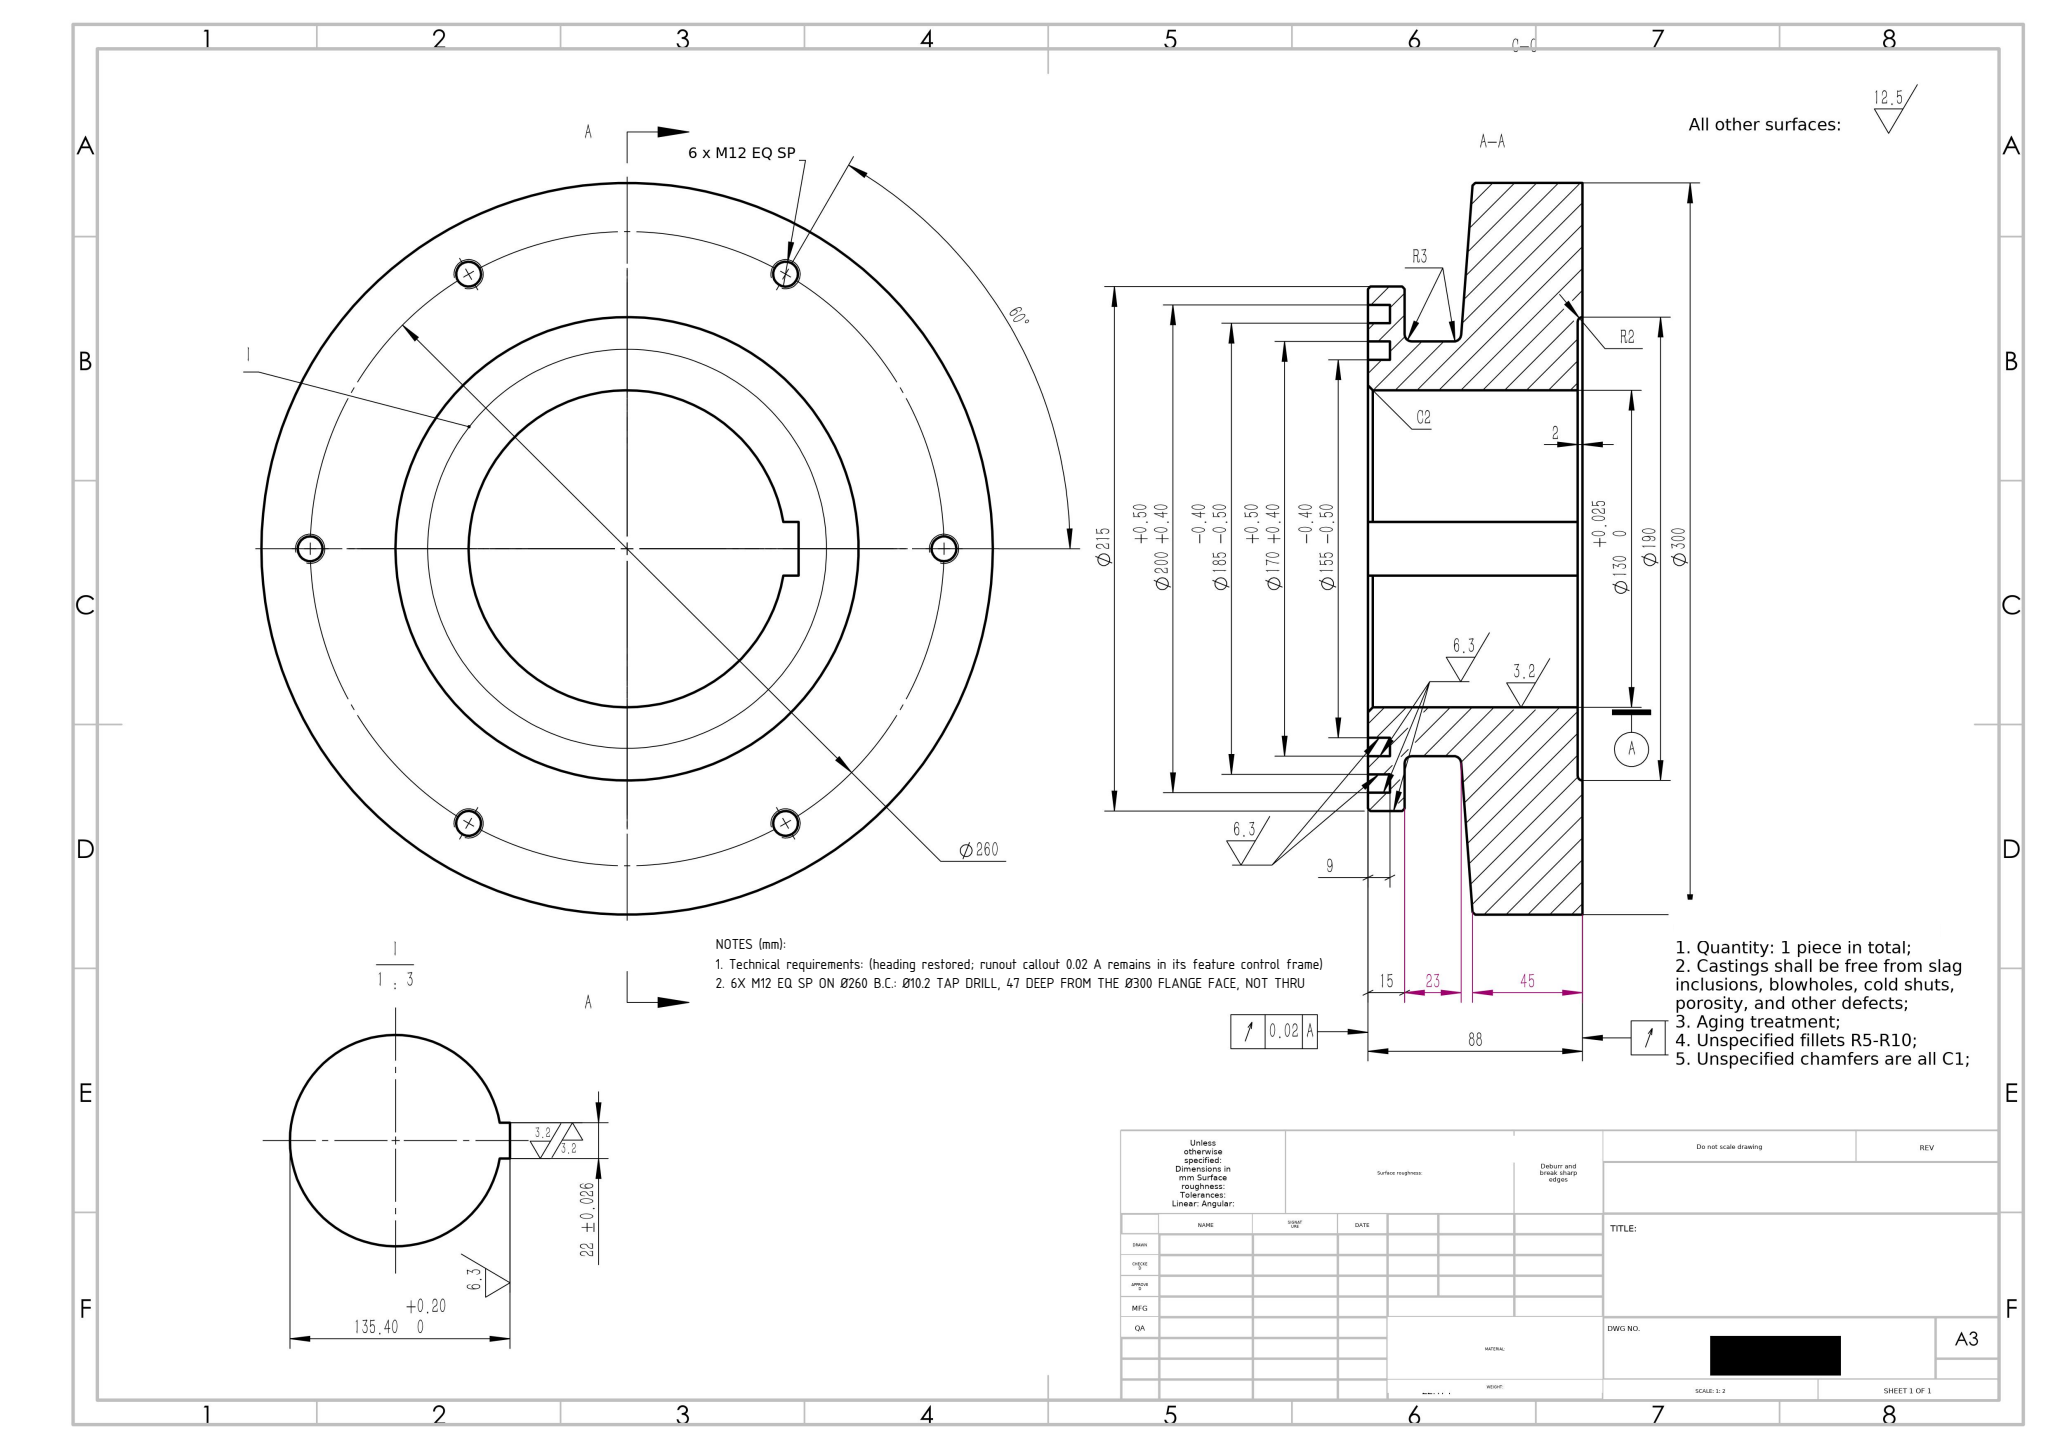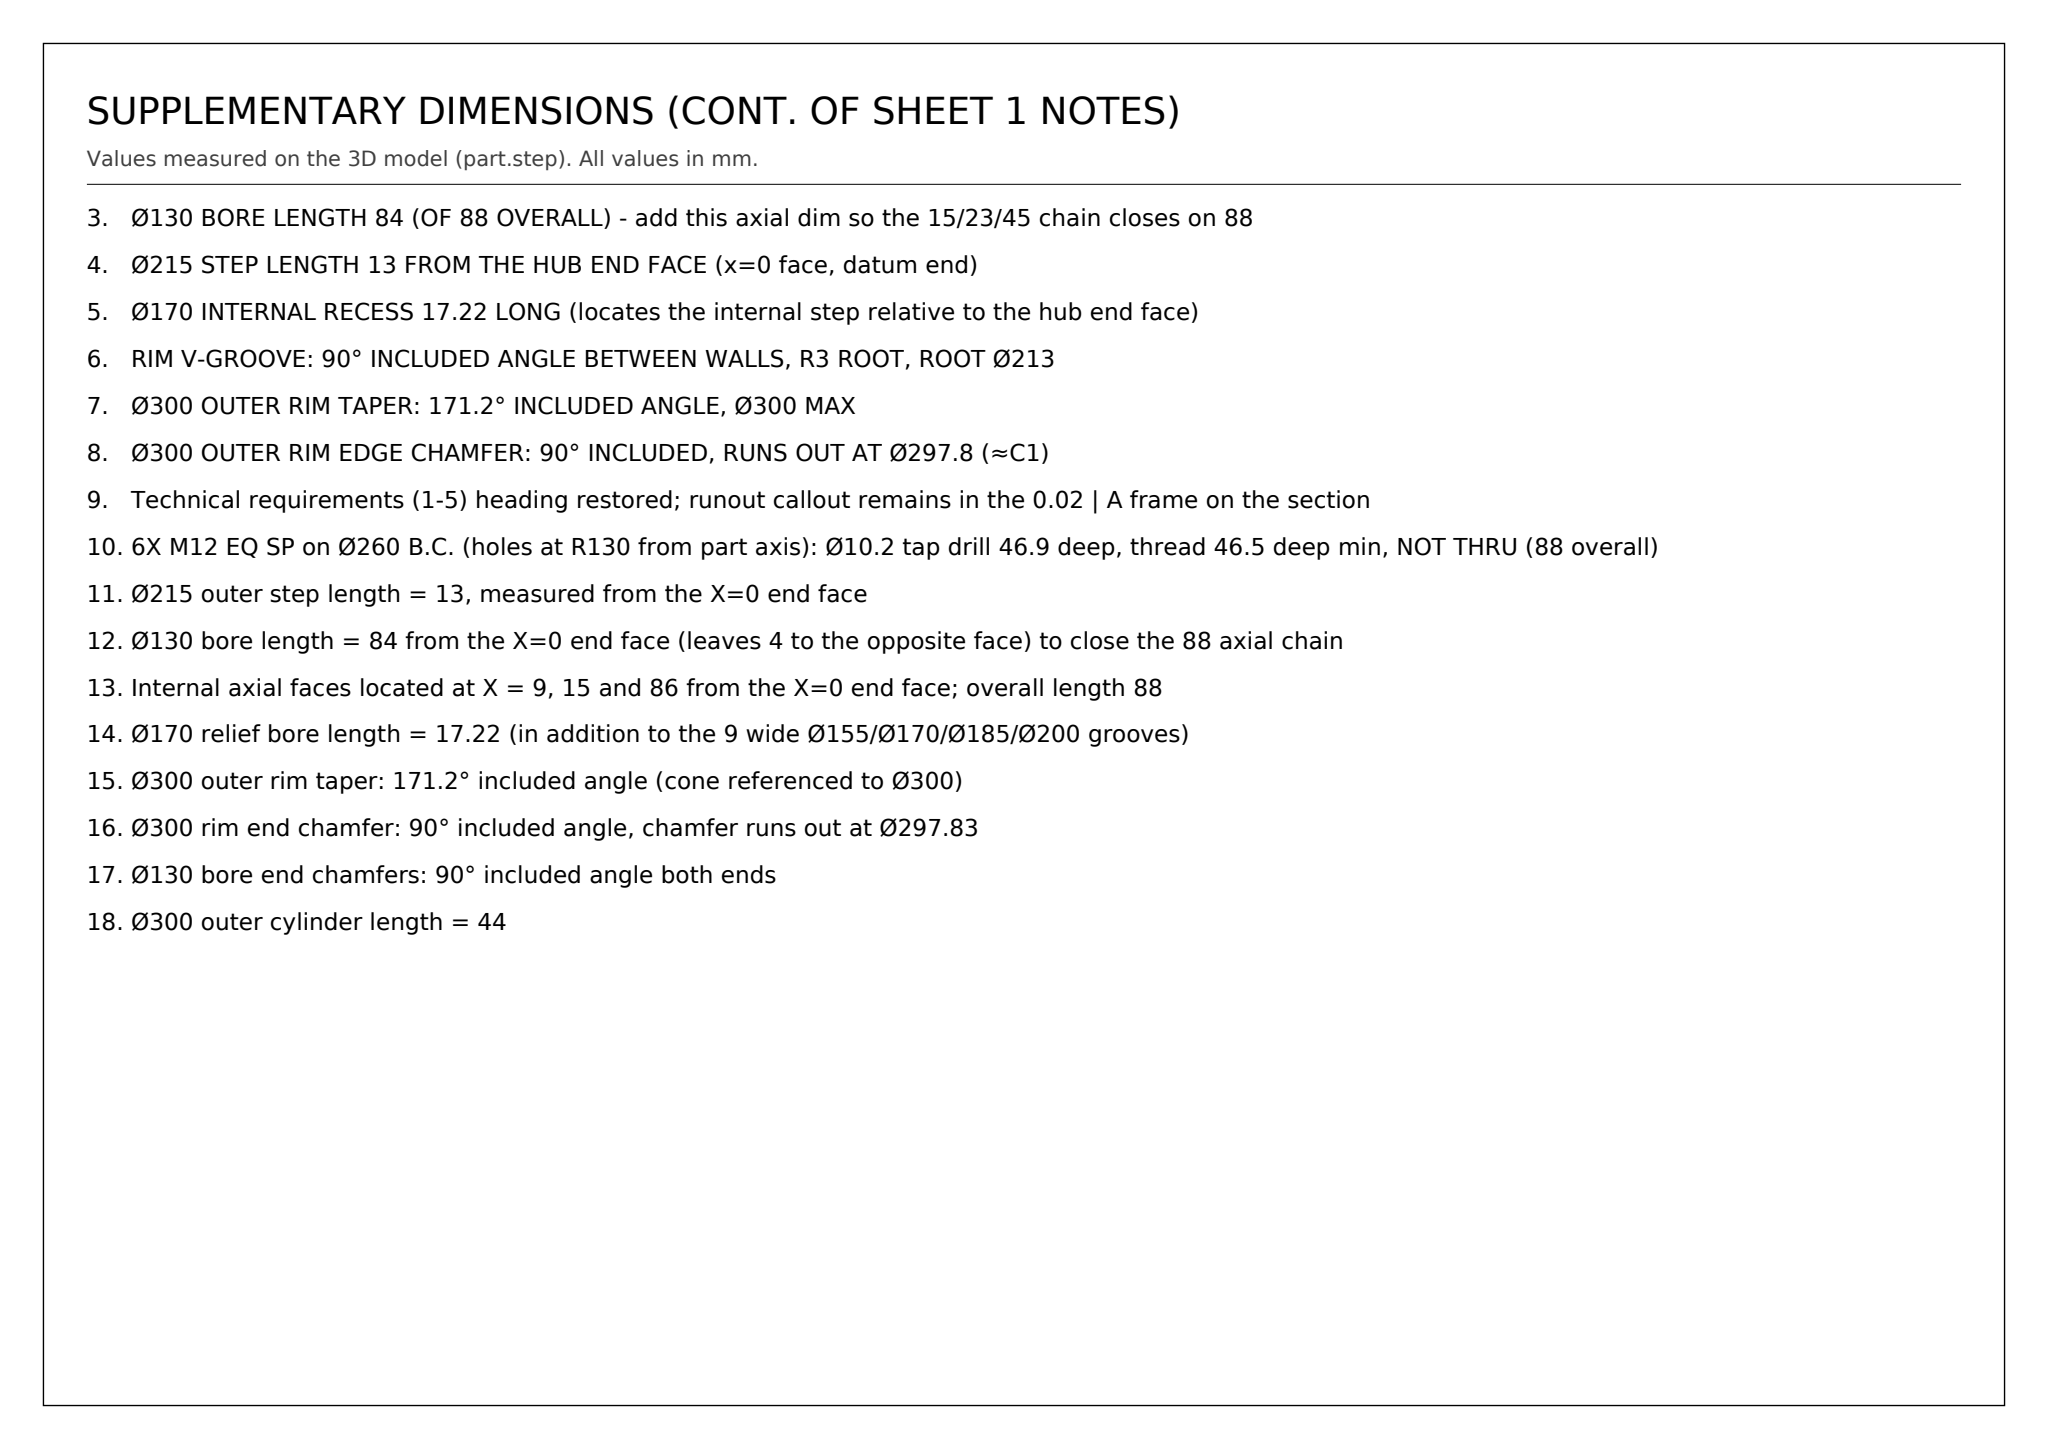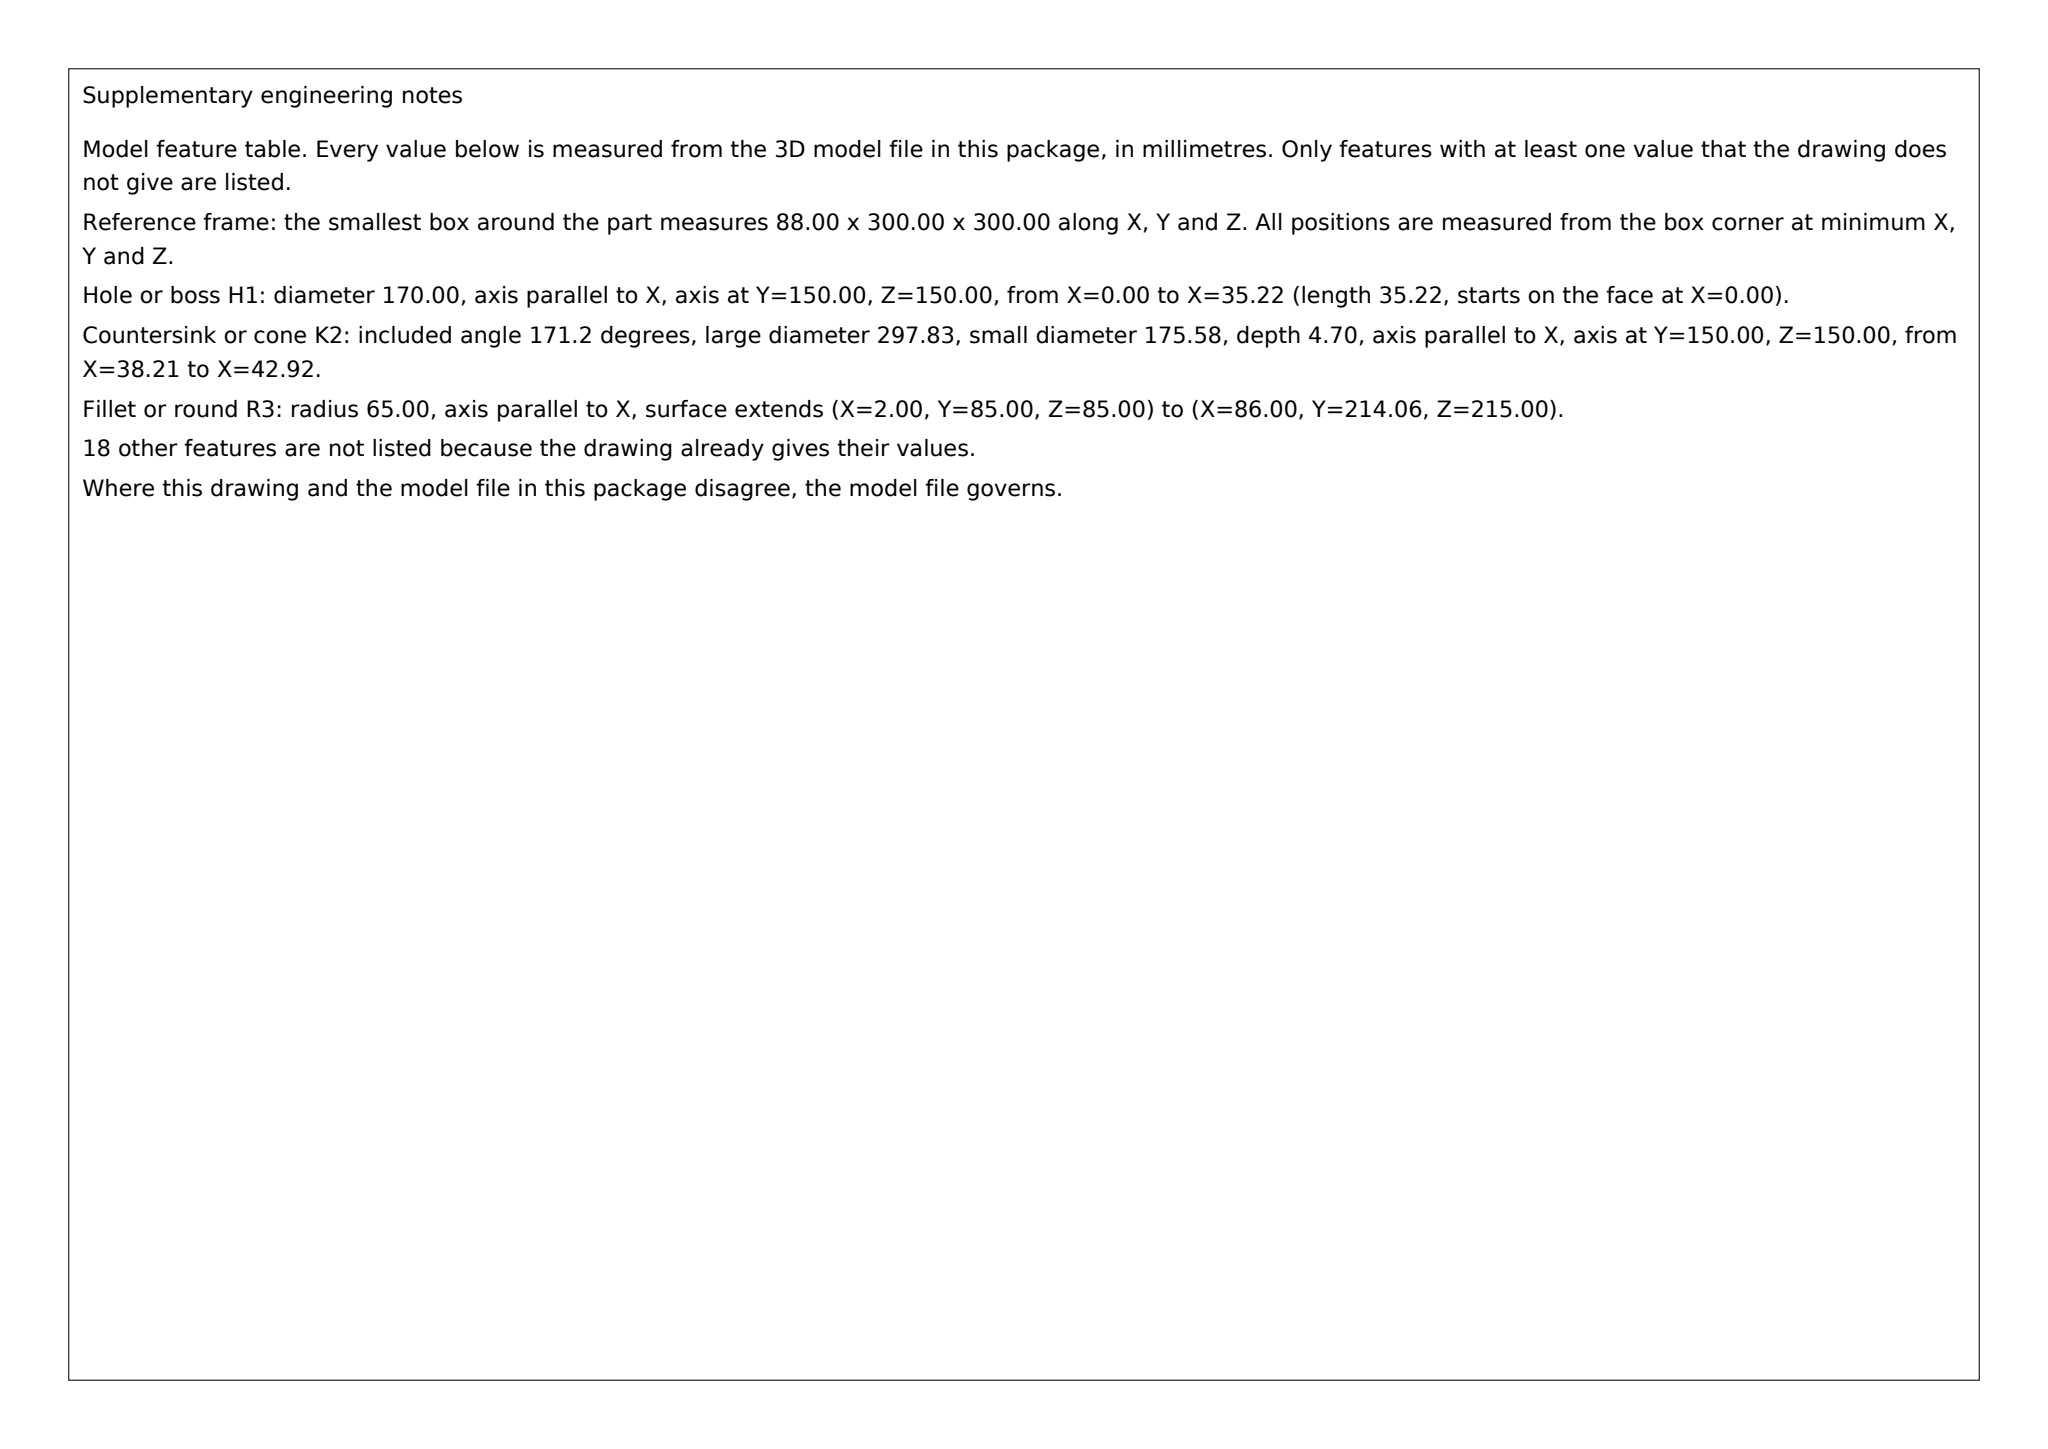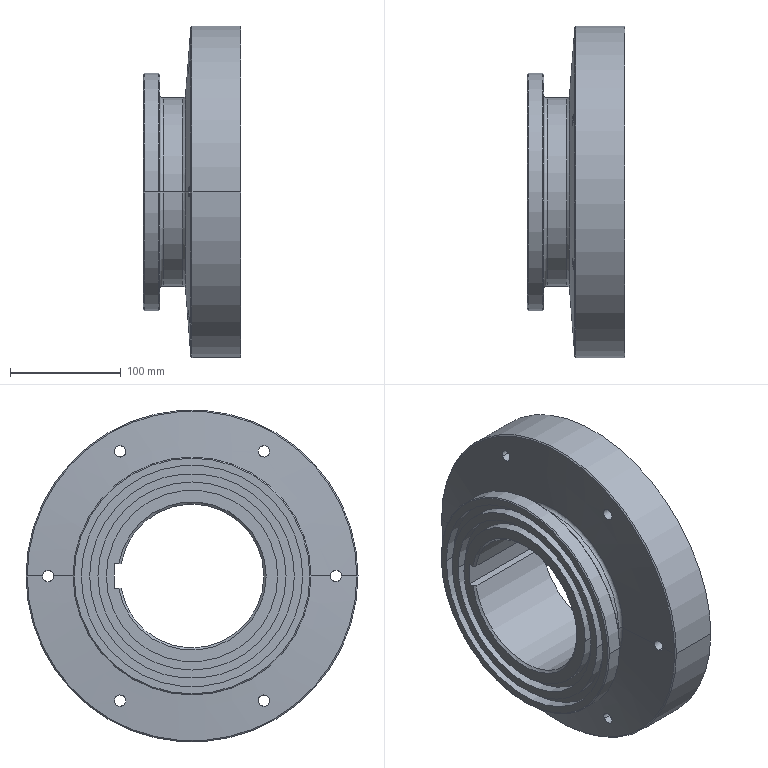Part | SolidWorks | mm | 1 solid | 55 faces | box 88 x 300 x 300 mm | volume 3163237 mm3 | cylinder 28 | plane 11 | cone 10 | torus 6 | commonest cylinder face diameters 10.2 x12 170 x4 200 x2 185 x2 155 x2 130 x2 300 x2 215 x2
Drawing notes:
Technical requirements: (heading restored; runout callout 0.02 A remains in its feature control frame) | from the solid: text overlap only - no STEP value lost
6X M12 EQ SP ON Ø260 B.C.: Ø10.2 TAP DRILL, 47 DEEP FROM THE Ø300 FLANGE FACE, NOT THRU | from the solid: cylinders[10.2,'x',...,46.93] x6 at radius 130 from axis (y150,z150)
Ø130 BORE LENGTH 84 (OF 88 OVERALL) - add this axial dim so the 15/23/45 chain closes on 88 | from the solid: cylinders[130.0,'x',[150,150],84.0]; bbox_xyz x=88
Ø215 STEP LENGTH 13 FROM THE HUB END FACE (x=0 face, datum end) | from the solid: cylinders[215.0,'x',[150,150],13.0]; axis_planes x=0.0
Ø170 INTERNAL RECESS 17.22 LONG (locates the internal step relative to the hub end face) | from the solid: cylinders[170.0,'x',[150,150],17.22]
RIM V-GROOVE: 90° INCLUDED ANGLE BETWEEN WALLS, R3 ROOT, ROOT Ø213 | from the solid: cones[90.0,215.0] and cones[90.0,213.0]; fillet_radii 3.0
Ø300 OUTER RIM TAPER: 171.2° INCLUDED ANGLE, Ø300 MAX | from the solid: cones[171.2,300.0]
Ø300 OUTER RIM EDGE CHAMFER: 90° INCLUDED, RUNS OUT AT Ø297.8 (≈C1) | from the solid: cones[90.0,297.833]
Technical requirements (1-5) heading restored; runout callout remains in the 0.02 | A frame on the section | from the solid: redaction of overlapping text block; no geometry value lost
6X M12 EQ SP on Ø260 B.C. (holes at R130 from part axis): Ø10.2 tap drill 46.9 deep, thread 46.5 deep min, NOT THRU (88 overall) | from the solid: cylinders[10.2,x] x12 at (y,z)=(20,150),(85,37.42),(85,262.58),(215,37.42),(215,262.58),(280,150), lengths 46.53/46.93; bbox_xyz x=88
Ø215 outer step length = 13, measured from the X=0 end face | from the solid: cylinders[215,x,(150,150),13]
Ø130 bore length = 84 from the X=0 end face (leaves 4 to the opposite face) to close the 88 axial chain | from the solid: cylinders[130,x,(150,150),84]; bbox x=88
Internal axial faces located at X = 9, 15 and 86 from the X=0 end face; overall length 88 | from the solid: axis_planes[x,0],[x,9],[x,15],[x,86],[x,88]
Ø170 relief bore length = 17.22 (in addition to the 9 wide Ø155/Ø170/Ø185/Ø200 grooves) | from the solid: cylinders[170,x,(150,150),17.22] vs cylinders[170,x,(150,150),9]
Ø300 outer rim taper: 171.2° included angle (cone referenced to Ø300) | from the solid: cones[171.2, ref_dia 300]
Ø300 rim end chamfer: 90° included angle, chamfer runs out at Ø297.83 | from the solid: cones[90.0, ref_dia 297.833]
Ø130 bore end chamfers: 90° included angle both ends | from the solid: cones[90.0, ref_dia 130] x2
Ø300 outer cylinder length = 44 | from the solid: cylinders[300,x,(150,150),44]